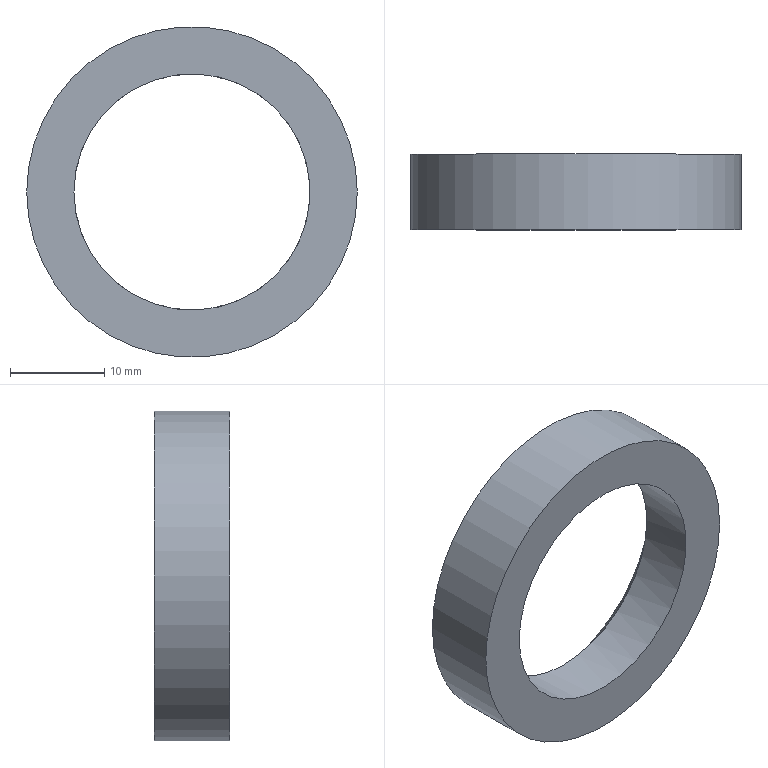Component | NX | SEALRING | 1 solid | 5 faces | box 35 x 8 x 35 mm | volume 3528 mm3 | cylinder 2 | plane 2 | sphere 1 | commonest cylinder face diameters 35 x1 25 x1
STEP:
#1=CARTESIAN_POINT('',(0.,0.,0.));
#2=DIRECTION('',(0.,0.,1.));
#3=DIRECTION('',(1.,0.,0.));
#4=AXIS2_PLACEMENT_3D('',#1,#2,#3);
#5=CARTESIAN_POINT('',(159.665,10.5,32.));
#6=VERTEX_POINT('',#5);
#7=CARTESIAN_POINT('',(177.165,10.5,32.));
#8=DIRECTION('',(0.,1.,0.));
#9=DIRECTION('',(-1.,0.,0.));
#10=AXIS2_PLACEMENT_3D('',#7,#8,#9);
#11=CIRCLE('',#10,17.5);
#12=CARTESIAN_POINT('',(177.165,10.5,32.));
#13=DIRECTION('',(0.,-1.,0.));
#14=DIRECTION('',(0.,0.,1.));
#15=AXIS2_PLACEMENT_3D('',#12,#13,#14);
#16=CYLINDRICAL_SURFACE('',#15,17.5);
#17=CARTESIAN_POINT('',(7.854,0.));
#18=DIRECTION('',(-1.,0.));
#19=VECTOR('',#18,1.);
#20=LINE('',#17,#19);
#21=(GEOMETRIC_REPRESENTATION_CONTEXT(2)PARAMETRIC_REPRESENTATION_CONTEXT()REPRESENTATION_CONTEXT('',''));
#22=DEFINITIONAL_REPRESENTATION('',(#20),#21);
#23=PCURVE('',#16,#22);
#24=CARTESIAN_POINT('',(177.165,10.5,32.));
#25=DIRECTION('',(0.,1.,0.));
#26=DIRECTION('',(0.,0.,-1.));
#27=AXIS2_PLACEMENT_3D('',#24,#25,#26);
#28=PLANE('',#27);
#29=CARTESIAN_POINT('',(0.,0.));
#30=DIRECTION('',(0.,1.));
#31=AXIS2_PLACEMENT_2D('',#29,#30);
#32=CIRCLE('',#31,17.5);
#33=(GEOMETRIC_REPRESENTATION_CONTEXT(2)PARAMETRIC_REPRESENTATION_CONTEXT()REPRESENTATION_CONTEXT('',''));
#34=DEFINITIONAL_REPRESENTATION('',(#32),#33);
#35=PCURVE('',#28,#34);
#36=SURFACE_CURVE('',#11,(#23,#35),.PCURVE_S1.);
#37=EDGE_CURVE('',#6,#6,#36,.T.);
#38=ORIENTED_EDGE('',*,*,#37,.F.);
#39=CARTESIAN_POINT('',(159.665,2.5,32.));
#40=VERTEX_POINT('',#39);
#41=CARTESIAN_POINT('',(159.665,10.5,32.));
#42=CARTESIAN_POINT('',(159.665,2.5,32.));
#43=B_SPLINE_CURVE_WITH_KNOTS('',1,(#41,#42),.UNSPECIFIED.,.F.,.F.,(2,2),(0.,8.),.PIECEWISE_BEZIER_KNOTS.);
#44=CARTESIAN_POINT('',(7.854,0.));
#45=DIRECTION('',(0.,1.));
#46=VECTOR('',#45,1.);
#47=LINE('',#44,#46);
#48=(GEOMETRIC_REPRESENTATION_CONTEXT(2)PARAMETRIC_REPRESENTATION_CONTEXT()REPRESENTATION_CONTEXT('',''));
#49=DEFINITIONAL_REPRESENTATION('',(#47),#48);
#50=PCURVE('',#16,#49);
#51=CARTESIAN_POINT('',(1.571,0.));
#52=DIRECTION('',(0.,1.));
#53=VECTOR('',#52,1.);
#54=LINE('',#51,#53);
#55=(GEOMETRIC_REPRESENTATION_CONTEXT(2)PARAMETRIC_REPRESENTATION_CONTEXT()REPRESENTATION_CONTEXT('',''));
#56=DEFINITIONAL_REPRESENTATION('',(#54),#55);
#57=PCURVE('',#16,#56);
#58=SEAM_CURVE('',#43,(#50,#57),.PCURVE_S1.);
#59=EDGE_CURVE('',#6,#40,#58,.T.);
#60=ORIENTED_EDGE('',*,*,#59,.T.);
#61=CARTESIAN_POINT('',(177.165,2.5,32.));
#62=DIRECTION('',(0.,1.,0.));
#63=DIRECTION('',(-1.,0.,0.));
#64=AXIS2_PLACEMENT_3D('',#61,#62,#63);
#65=CIRCLE('',#64,17.5);
#66=CARTESIAN_POINT('',(7.854,8.));
#67=DIRECTION('',(-1.,0.));
#68=VECTOR('',#67,1.);
#69=LINE('',#66,#68);
#70=(GEOMETRIC_REPRESENTATION_CONTEXT(2)PARAMETRIC_REPRESENTATION_CONTEXT()REPRESENTATION_CONTEXT('',''));
#71=DEFINITIONAL_REPRESENTATION('',(#69),#70);
#72=PCURVE('',#16,#71);
#73=CARTESIAN_POINT('',(177.165,2.5,32.));
#74=DIRECTION('',(0.,1.,0.));
#75=DIRECTION('',(0.,0.,-1.));
#76=AXIS2_PLACEMENT_3D('',#73,#74,#75);
#77=PLANE('',#76);
#78=CARTESIAN_POINT('',(0.,0.));
#79=DIRECTION('',(0.,1.));
#80=AXIS2_PLACEMENT_2D('',#78,#79);
#81=CIRCLE('',#80,17.5);
#82=(GEOMETRIC_REPRESENTATION_CONTEXT(2)PARAMETRIC_REPRESENTATION_CONTEXT()REPRESENTATION_CONTEXT('',''));
#83=DEFINITIONAL_REPRESENTATION('',(#81),#82);
#84=PCURVE('',#77,#83);
#85=SURFACE_CURVE('',#65,(#72,#84),.PCURVE_S1.);
#86=EDGE_CURVE('',#40,#40,#85,.T.);
#87=ORIENTED_EDGE('',*,*,#86,.T.);
#88=ORIENTED_EDGE('',*,*,#59,.F.);
#89=EDGE_LOOP('',(#38,#60,#87,#88));
#90=FACE_BOUND('',#89,.T.);
#91=ADVANCED_FACE('',(#90),#16,.T.);
#92=CARTESIAN_POINT('',(177.165,8.396,19.5));
#93=VERTEX_POINT('',#92);
#94=CARTESIAN_POINT('',(164.665,8.396,32.));
#95=VERTEX_POINT('',#94);
#96=CARTESIAN_POINT('',(177.165,8.396,32.));
#97=DIRECTION('',(0.,-1.,0.));
#98=DIRECTION('',(0.,0.,-1.));
#99=AXIS2_PLACEMENT_3D('',#96,#97,#98);
#100=CIRCLE('',#99,12.5);
#101=CARTESIAN_POINT('',(177.165,10.5,32.));
#102=DIRECTION('',(0.,-1.,0.));
#103=DIRECTION('',(0.,0.,1.));
#104=AXIS2_PLACEMENT_3D('',#101,#102,#103);
#105=CYLINDRICAL_SURFACE('',#104,12.5);
#106=CARTESIAN_POINT('',(3.142,2.104));
#107=DIRECTION('',(1.,0.));
#108=VECTOR('',#107,1.);
#109=LINE('',#106,#108);
#110=(GEOMETRIC_REPRESENTATION_CONTEXT(2)PARAMETRIC_REPRESENTATION_CONTEXT()REPRESENTATION_CONTEXT('',''));
#111=DEFINITIONAL_REPRESENTATION('',(#109),#110);
#112=PCURVE('',#105,#111);
#113=CARTESIAN_POINT('',(177.165,26.5,32.));
#114=DIRECTION('',(0.,0.,1.));
#115=DIRECTION('',(-1.,0.,0.));
#116=AXIS2_PLACEMENT_3D('',#113,#114,#115);
#117=SPHERICAL_SURFACE('',#116,22.);
#118=CARTESIAN_POINT('',(1.571,-0.6043));
#119=CARTESIAN_POINT('',(1.62,-0.6045));
#120=CARTESIAN_POINT('',(1.718,-0.5935));
#121=CARTESIAN_POINT('',(1.854,-0.5475));
#122=CARTESIAN_POINT('',(1.967,-0.4755));
#123=CARTESIAN_POINT('',(2.056,-0.3837));
#124=CARTESIAN_POINT('',(2.12,-0.2774));
#125=CARTESIAN_POINT('',(2.16,-0.1616));
#126=CARTESIAN_POINT('',(2.177,-0.04075));
#127=CARTESIAN_POINT('',(2.174,0.08137));
#128=CARTESIAN_POINT('',(2.149,0.201));
#129=CARTESIAN_POINT('',(2.101,0.3141));
#130=CARTESIAN_POINT('',(2.029,0.4161));
#131=CARTESIAN_POINT('',(1.932,0.502));
#132=CARTESIAN_POINT('',(1.811,0.566));
#133=CARTESIAN_POINT('',(1.67,0.6025));
#134=CARTESIAN_POINT('',(1.521,0.6078));
#135=CARTESIAN_POINT('',(1.376,0.5814));
#136=CARTESIAN_POINT('',(1.247,0.5261));
#137=CARTESIAN_POINT('',(1.142,0.4468));
#138=CARTESIAN_POINT('',(1.062,0.3496));
#139=CARTESIAN_POINT('',(1.006,0.2396));
#140=CARTESIAN_POINT('',(0.9736,0.1217));
#141=CARTESIAN_POINT('',(0.9666,0.04054));
#142=CARTESIAN_POINT('',(0.9665,0.));
#143=B_SPLINE_CURVE_WITH_KNOTS('',3,(#118,#119,#120,#121,#122,#123,#124,#125,#126,#127,#128,#129,#130,#131,#132,#133,#134,#135,#136,#137,#138,#139,#140,#141,#142),.UNSPECIFIED.,.F.,.F.,(4,1,1,1,1,1,1,1,1,1,1,1,1,1,1,1,1,1,1,1,1,1,4),(0.,0.2142,0.4284,0.6426,0.8568,1.071,1.285,1.499,1.714,1.928,2.142,2.356,2.57,2.785,2.999,3.213,3.427,3.641,3.856,4.07,4.284,4.498,4.712),.QUASI_UNIFORM_KNOTS.);
#144=(GEOMETRIC_REPRESENTATION_CONTEXT(2)PARAMETRIC_REPRESENTATION_CONTEXT()REPRESENTATION_CONTEXT('',''));
#145=DEFINITIONAL_REPRESENTATION('',(#143),#144);
#146=PCURVE('',#117,#145);
#147=SURFACE_CURVE('',#100,(#112,#146),.PCURVE_S1.);
#148=EDGE_CURVE('',#93,#95,#147,.T.);
#149=ORIENTED_EDGE('',*,*,#148,.T.);
#150=CARTESIAN_POINT('',(164.665,2.5,32.));
#151=VERTEX_POINT('',#150);
#152=CARTESIAN_POINT('',(164.665,8.396,32.));
#153=CARTESIAN_POINT('',(164.665,2.5,32.));
#154=B_SPLINE_CURVE_WITH_KNOTS('',1,(#152,#153),.UNSPECIFIED.,.F.,.F.,(2,2),(2.104,8.),.PIECEWISE_BEZIER_KNOTS.);
#155=CARTESIAN_POINT('',(7.854,0.));
#156=DIRECTION('',(0.,1.));
#157=VECTOR('',#156,1.);
#158=LINE('',#155,#157);
#159=(GEOMETRIC_REPRESENTATION_CONTEXT(2)PARAMETRIC_REPRESENTATION_CONTEXT()REPRESENTATION_CONTEXT('',''));
#160=DEFINITIONAL_REPRESENTATION('',(#158),#159);
#161=PCURVE('',#105,#160);
#162=CARTESIAN_POINT('',(1.571,0.));
#163=DIRECTION('',(0.,1.));
#164=VECTOR('',#163,1.);
#165=LINE('',#162,#164);
#166=(GEOMETRIC_REPRESENTATION_CONTEXT(2)PARAMETRIC_REPRESENTATION_CONTEXT()REPRESENTATION_CONTEXT('',''));
#167=DEFINITIONAL_REPRESENTATION('',(#165),#166);
#168=PCURVE('',#105,#167);
#169=SEAM_CURVE('',#154,(#161,#168),.PCURVE_S1.);
#170=EDGE_CURVE('',#95,#151,#169,.T.);
#171=ORIENTED_EDGE('',*,*,#170,.T.);
#172=CARTESIAN_POINT('',(177.165,2.5,32.));
#173=DIRECTION('',(0.,1.,0.));
#174=DIRECTION('',(-1.,0.,0.));
#175=AXIS2_PLACEMENT_3D('',#172,#173,#174);
#176=CIRCLE('',#175,12.5);
#177=CARTESIAN_POINT('',(7.854,8.));
#178=DIRECTION('',(-1.,0.));
#179=VECTOR('',#178,1.);
#180=LINE('',#177,#179);
#181=(GEOMETRIC_REPRESENTATION_CONTEXT(2)PARAMETRIC_REPRESENTATION_CONTEXT()REPRESENTATION_CONTEXT('',''));
#182=DEFINITIONAL_REPRESENTATION('',(#180),#181);
#183=PCURVE('',#105,#182);
#184=CARTESIAN_POINT('',(0.,0.));
#185=DIRECTION('',(0.,1.));
#186=AXIS2_PLACEMENT_2D('',#184,#185);
#187=CIRCLE('',#186,12.5);
#188=(GEOMETRIC_REPRESENTATION_CONTEXT(2)PARAMETRIC_REPRESENTATION_CONTEXT()REPRESENTATION_CONTEXT('',''));
#189=DEFINITIONAL_REPRESENTATION('',(#187),#188);
#190=PCURVE('',#77,#189);
#191=SURFACE_CURVE('',#176,(#183,#190),.PCURVE_S1.);
#192=EDGE_CURVE('',#151,#151,#191,.T.);
#193=ORIENTED_EDGE('',*,*,#192,.T.);
#194=ORIENTED_EDGE('',*,*,#170,.F.);
#195=CARTESIAN_POINT('',(177.165,8.396,32.));
#196=DIRECTION('',(0.,-1.,0.));
#197=DIRECTION('',(0.,0.,-1.));
#198=AXIS2_PLACEMENT_3D('',#195,#196,#197);
#199=CIRCLE('',#198,12.5);
#200=CARTESIAN_POINT('',(-3.142,2.104));
#201=DIRECTION('',(1.,0.));
#202=VECTOR('',#201,1.);
#203=LINE('',#200,#202);
#204=(GEOMETRIC_REPRESENTATION_CONTEXT(2)PARAMETRIC_REPRESENTATION_CONTEXT()REPRESENTATION_CONTEXT('',''));
#205=DEFINITIONAL_REPRESENTATION('',(#203),#204);
#206=PCURVE('',#105,#205);
#207=CARTESIAN_POINT('',(0.9665,0.));
#208=CARTESIAN_POINT('',(0.9665,-0.01352));
#209=CARTESIAN_POINT('',(0.9673,-0.04057));
#210=CARTESIAN_POINT('',(0.9709,-0.081));
#211=CARTESIAN_POINT('',(0.9769,-0.1211));
#212=CARTESIAN_POINT('',(0.9853,-0.1609));
#213=CARTESIAN_POINT('',(0.9962,-0.2));
#214=CARTESIAN_POINT('',(1.01,-0.2384));
#215=CARTESIAN_POINT('',(1.026,-0.276));
#216=CARTESIAN_POINT('',(1.044,-0.3124));
#217=CARTESIAN_POINT('',(1.065,-0.3477));
#218=CARTESIAN_POINT('',(1.089,-0.3815));
#219=CARTESIAN_POINT('',(1.116,-0.4137));
#220=CARTESIAN_POINT('',(1.146,-0.4442));
#221=CARTESIAN_POINT('',(1.178,-0.4726));
#222=CARTESIAN_POINT('',(1.213,-0.4988));
#223=CARTESIAN_POINT('',(1.251,-0.5225));
#224=CARTESIAN_POINT('',(1.291,-0.5436));
#225=CARTESIAN_POINT('',(1.334,-0.5619));
#226=CARTESIAN_POINT('',(1.378,-0.5771));
#227=CARTESIAN_POINT('',(1.425,-0.5892));
#228=CARTESIAN_POINT('',(1.473,-0.5979));
#229=CARTESIAN_POINT('',(1.521,-0.6031));
#230=CARTESIAN_POINT('',(1.554,-0.6043));
#231=CARTESIAN_POINT('',(1.571,-0.6043));
#232=B_SPLINE_CURVE_WITH_KNOTS('',3,(#207,#208,#209,#210,#211,#212,#213,#214,#215,#216,#217,#218,#219,#220,#221,#222,#223,#224,#225,#226,#227,#228,#229,#230,#231),.UNSPECIFIED.,.F.,.F.,(4,1,1,1,1,1,1,1,1,1,1,1,1,1,1,1,1,1,1,1,1,1,4),(4.712,4.784,4.855,4.927,4.998,5.069,5.141,5.212,5.284,5.355,5.426,5.498,5.569,5.641,5.712,5.783,5.855,5.926,5.998,6.069,6.14,6.212,6.283),.QUASI_UNIFORM_KNOTS.);
#233=(GEOMETRIC_REPRESENTATION_CONTEXT(2)PARAMETRIC_REPRESENTATION_CONTEXT()REPRESENTATION_CONTEXT('',''));
#234=DEFINITIONAL_REPRESENTATION('',(#232),#233);
#235=PCURVE('',#117,#234);
#236=SURFACE_CURVE('',#199,(#206,#235),.PCURVE_S1.);
#237=EDGE_CURVE('',#95,#93,#236,.T.);
#238=ORIENTED_EDGE('',*,*,#237,.T.);
#239=EDGE_LOOP('',(#149,#171,#193,#194,#238));
#240=FACE_BOUND('',#239,.F.);
#241=ADVANCED_FACE('',(#240),#105,.F.);
#242=CARTESIAN_POINT('',(177.165,10.5,16.9));
#243=VERTEX_POINT('',#242);
#244=CARTESIAN_POINT('',(177.165,10.5,32.));
#245=DIRECTION('',(0.,1.,0.));
#246=DIRECTION('',(0.,0.,-1.));
#247=AXIS2_PLACEMENT_3D('',#244,#245,#246);
#248=CIRCLE('',#247,15.1);
#249=CARTESIAN_POINT('',(0.,0.));
#250=DIRECTION('',(1.,0.));
#251=AXIS2_PLACEMENT_2D('',#249,#250);
#252=CIRCLE('',#251,15.1);
#253=(GEOMETRIC_REPRESENTATION_CONTEXT(2)PARAMETRIC_REPRESENTATION_CONTEXT()REPRESENTATION_CONTEXT('',''));
#254=DEFINITIONAL_REPRESENTATION('',(#252),#253);
#255=PCURVE('',#28,#254);
#256=CARTESIAN_POINT('',(1.571,-0.7565));
#257=CARTESIAN_POINT('',(1.478,-0.7571));
#258=CARTESIAN_POINT('',(1.303,-0.7299));
#259=CARTESIAN_POINT('',(1.087,-0.6232));
#260=CARTESIAN_POINT('',(0.9417,-0.4706));
#261=CARTESIAN_POINT('',(0.8536,-0.2914));
#262=CARTESIAN_POINT('',(0.8126,-0.09853));
#263=CARTESIAN_POINT('',(0.8126,0.09853));
#264=CARTESIAN_POINT('',(0.8536,0.2914));
#265=CARTESIAN_POINT('',(0.9416,0.4706));
#266=CARTESIAN_POINT('',(1.088,0.6231));
#267=CARTESIAN_POINT('',(1.302,0.7301));
#268=CARTESIAN_POINT('',(1.571,0.7696));
#269=CARTESIAN_POINT('',(1.84,0.7301));
#270=CARTESIAN_POINT('',(2.054,0.6231));
#271=CARTESIAN_POINT('',(2.2,0.4706));
#272=CARTESIAN_POINT('',(2.288,0.2914));
#273=CARTESIAN_POINT('',(2.329,0.09853));
#274=CARTESIAN_POINT('',(2.329,-0.09853));
#275=CARTESIAN_POINT('',(2.288,-0.2914));
#276=CARTESIAN_POINT('',(2.2,-0.4706));
#277=CARTESIAN_POINT('',(2.054,-0.6232));
#278=CARTESIAN_POINT('',(1.838,-0.7299));
#279=CARTESIAN_POINT('',(1.664,-0.7571));
#280=CARTESIAN_POINT('',(1.571,-0.7565));
#281=B_SPLINE_CURVE_WITH_KNOTS('',3,(#256,#257,#258,#259,#260,#261,#262,#263,#264,#265,#266,#267,#268,#269,#270,#271,#272,#273,#274,#275,#276,#277,#278,#279,#280),.UNSPECIFIED.,.T.,.F.,(4,1,1,1,1,1,1,1,1,1,1,1,1,1,1,1,1,1,1,1,1,1,4),(0.,0.2856,0.5712,0.8568,1.142,1.428,1.714,1.999,2.285,2.57,2.856,3.142,3.427,3.713,3.998,4.284,4.57,4.855,5.141,5.426,5.712,5.998,6.283),.QUASI_UNIFORM_KNOTS.);
#282=(GEOMETRIC_REPRESENTATION_CONTEXT(2)PARAMETRIC_REPRESENTATION_CONTEXT()REPRESENTATION_CONTEXT('',''));
#283=DEFINITIONAL_REPRESENTATION('',(#281),#282);
#284=PCURVE('',#117,#283);
#285=SURFACE_CURVE('',#248,(#255,#284),.PCURVE_S1.);
#286=EDGE_CURVE('',#243,#243,#285,.T.);
#287=ORIENTED_EDGE('',*,*,#286,.F.);
#288=EDGE_LOOP('',(#287));
#289=FACE_BOUND('',#288,.T.);
#290=ORIENTED_EDGE('',*,*,#37,.T.);
#291=EDGE_LOOP('',(#290));
#292=FACE_BOUND('',#291,.T.);
#293=ADVANCED_FACE('',(#289,#292),#28,.T.);
#294=ORIENTED_EDGE('',*,*,#86,.F.);
#295=EDGE_LOOP('',(#294));
#296=FACE_BOUND('',#295,.T.);
#297=ORIENTED_EDGE('',*,*,#192,.T.);
#298=EDGE_LOOP('',(#297));
#299=FACE_BOUND('',#298,.T.);
#300=ADVANCED_FACE('',(#296,#299),#77,.F.);
#301=ORIENTED_EDGE('',*,*,#237,.F.);
#302=ORIENTED_EDGE('',*,*,#148,.F.);
#303=EDGE_LOOP('',(#301,#302));
#304=FACE_BOUND('',#303,.F.);
#305=ORIENTED_EDGE('',*,*,#286,.F.);
#306=EDGE_LOOP('',(#305));
#307=FACE_BOUND('',#306,.F.);
#308=ADVANCED_FACE('',(#304,#307),#117,.F.);
#309=CLOSED_SHELL('',(#91,#241,#293,#300,#308));
#310=MANIFOLD_SOLID_BREP('',#309);
#311=(LENGTH_UNIT()NAMED_UNIT(*)SI_UNIT(.MILLI.,.METRE.));
#312=UNCERTAINTY_MEASURE_WITH_UNIT(LENGTH_MEASURE(0.000005),#311,'','');
#313=(NAMED_UNIT(*)PLANE_ANGLE_UNIT()SI_UNIT($,.RADIAN.));
#314=(NAMED_UNIT(*)SI_UNIT($,.STERADIAN.)SOLID_ANGLE_UNIT());
#315=(GEOMETRIC_REPRESENTATION_CONTEXT(3)GLOBAL_UNCERTAINTY_ASSIGNED_CONTEXT((#312))GLOBAL_UNIT_ASSIGNED_CONTEXT((#311,#313,#314))REPRESENTATION_CONTEXT('',''));
#316=ADVANCED_BREP_SHAPE_REPRESENTATION('',(#4,#310),#315);